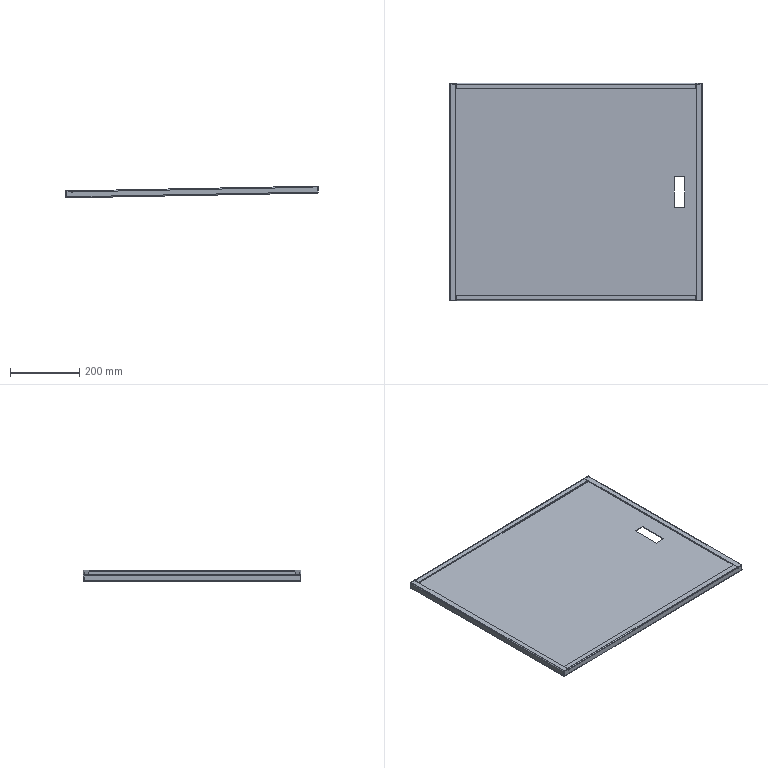Component | SolidWorks | 11BottomDoor-4 | 1 solid | 102 faces | volume 1074206 mm3 | plane 78 | cylinder 24 | commonest cylinder face diameters 4.2 x8 6 x8 2 x8 | material A3 Steel